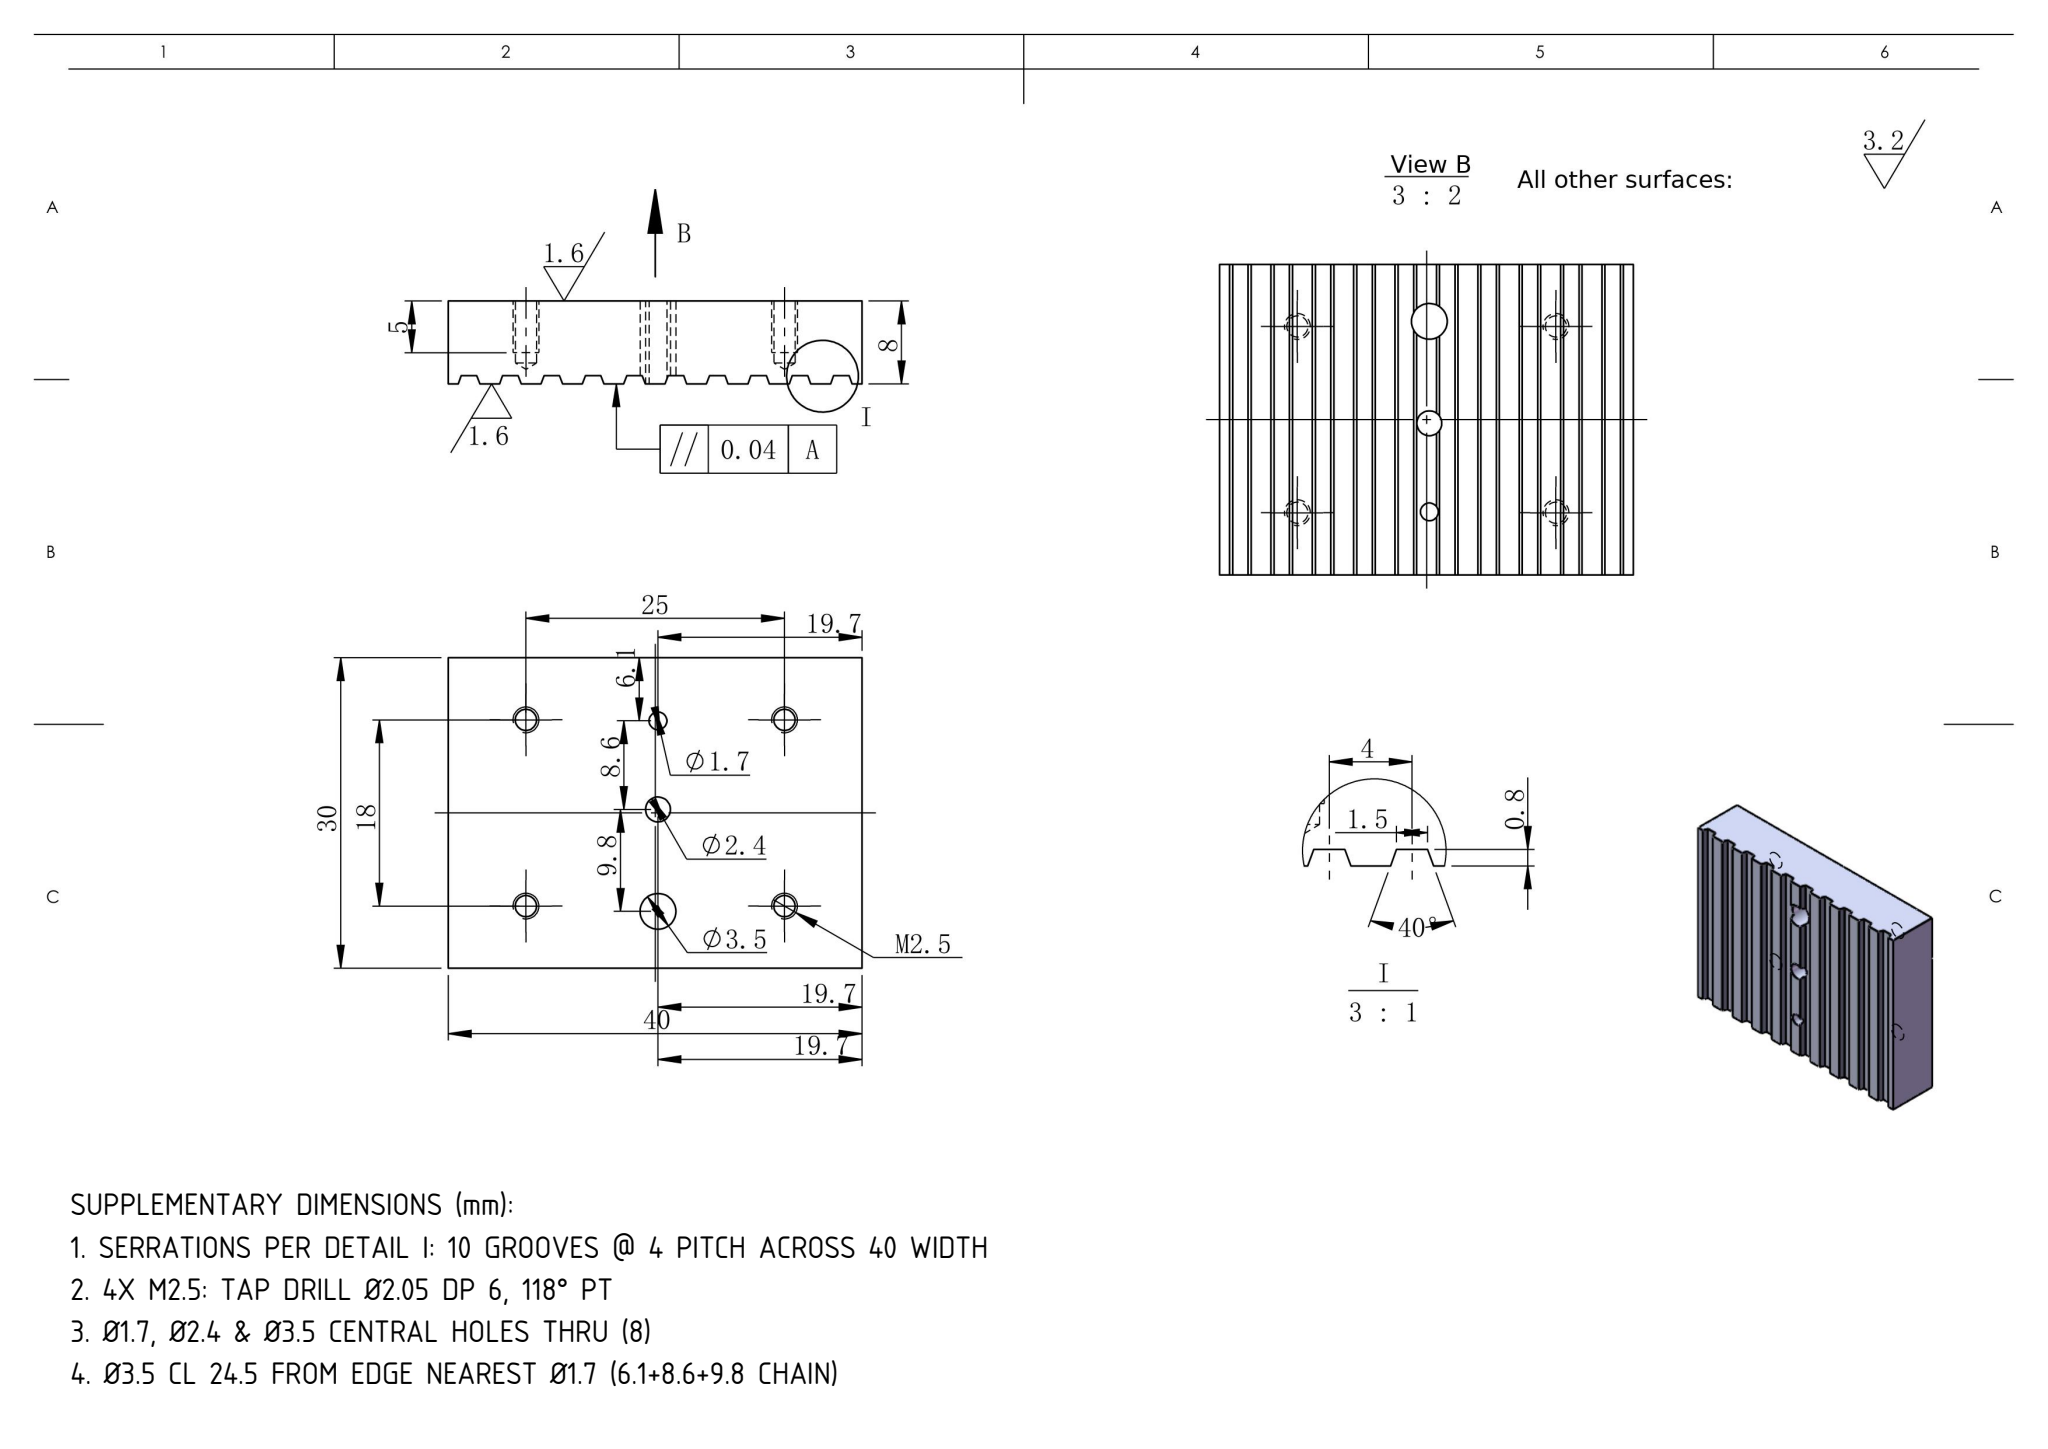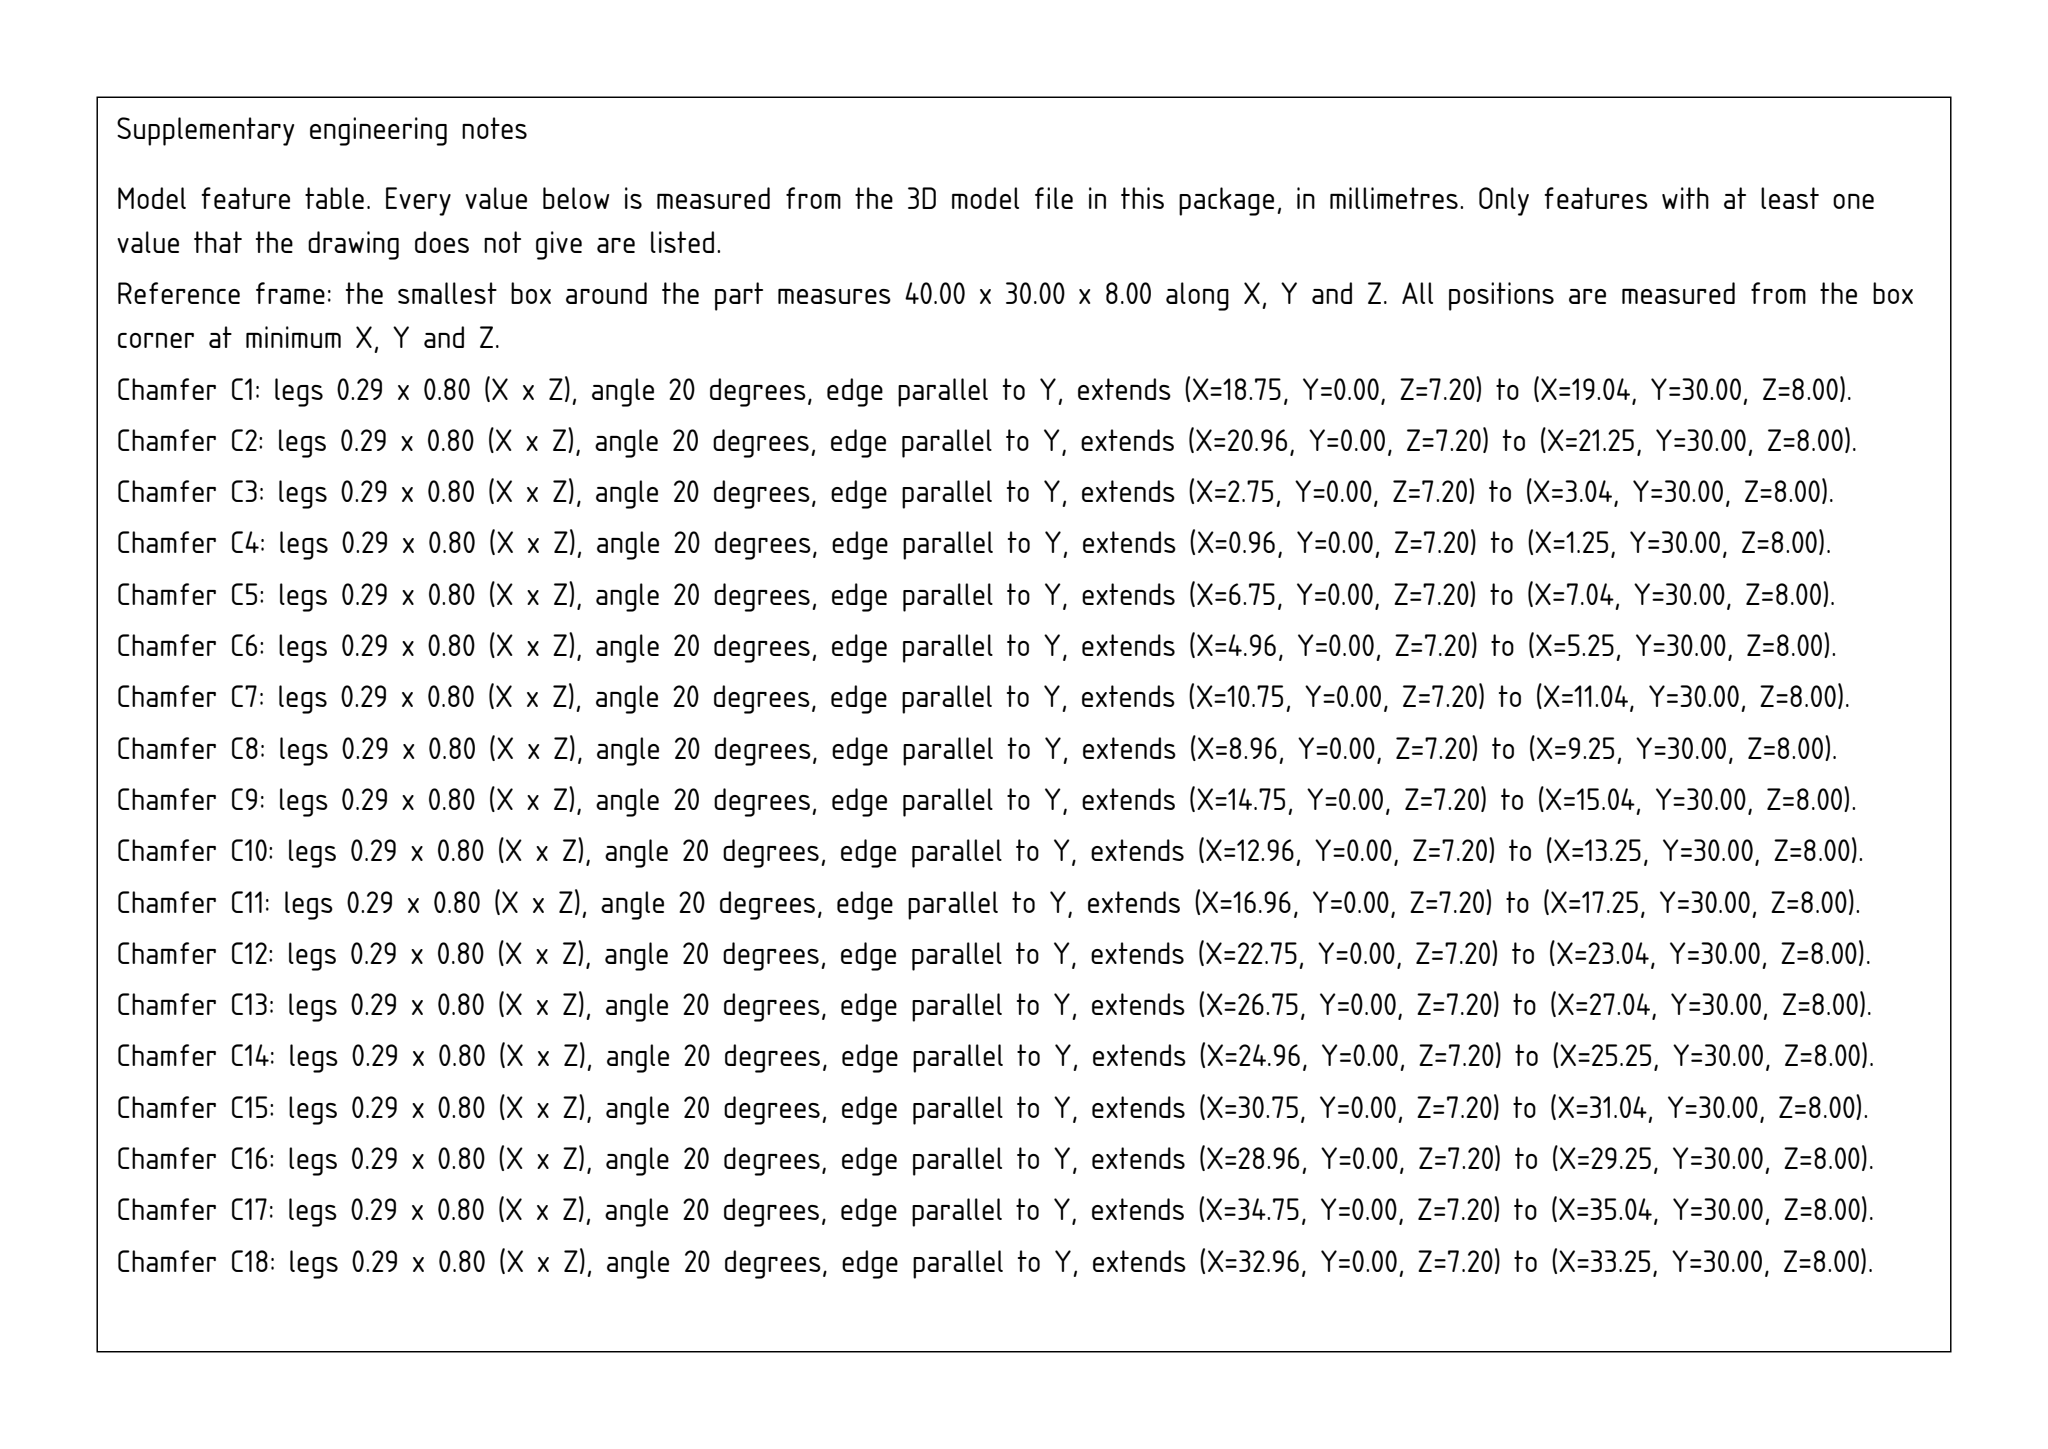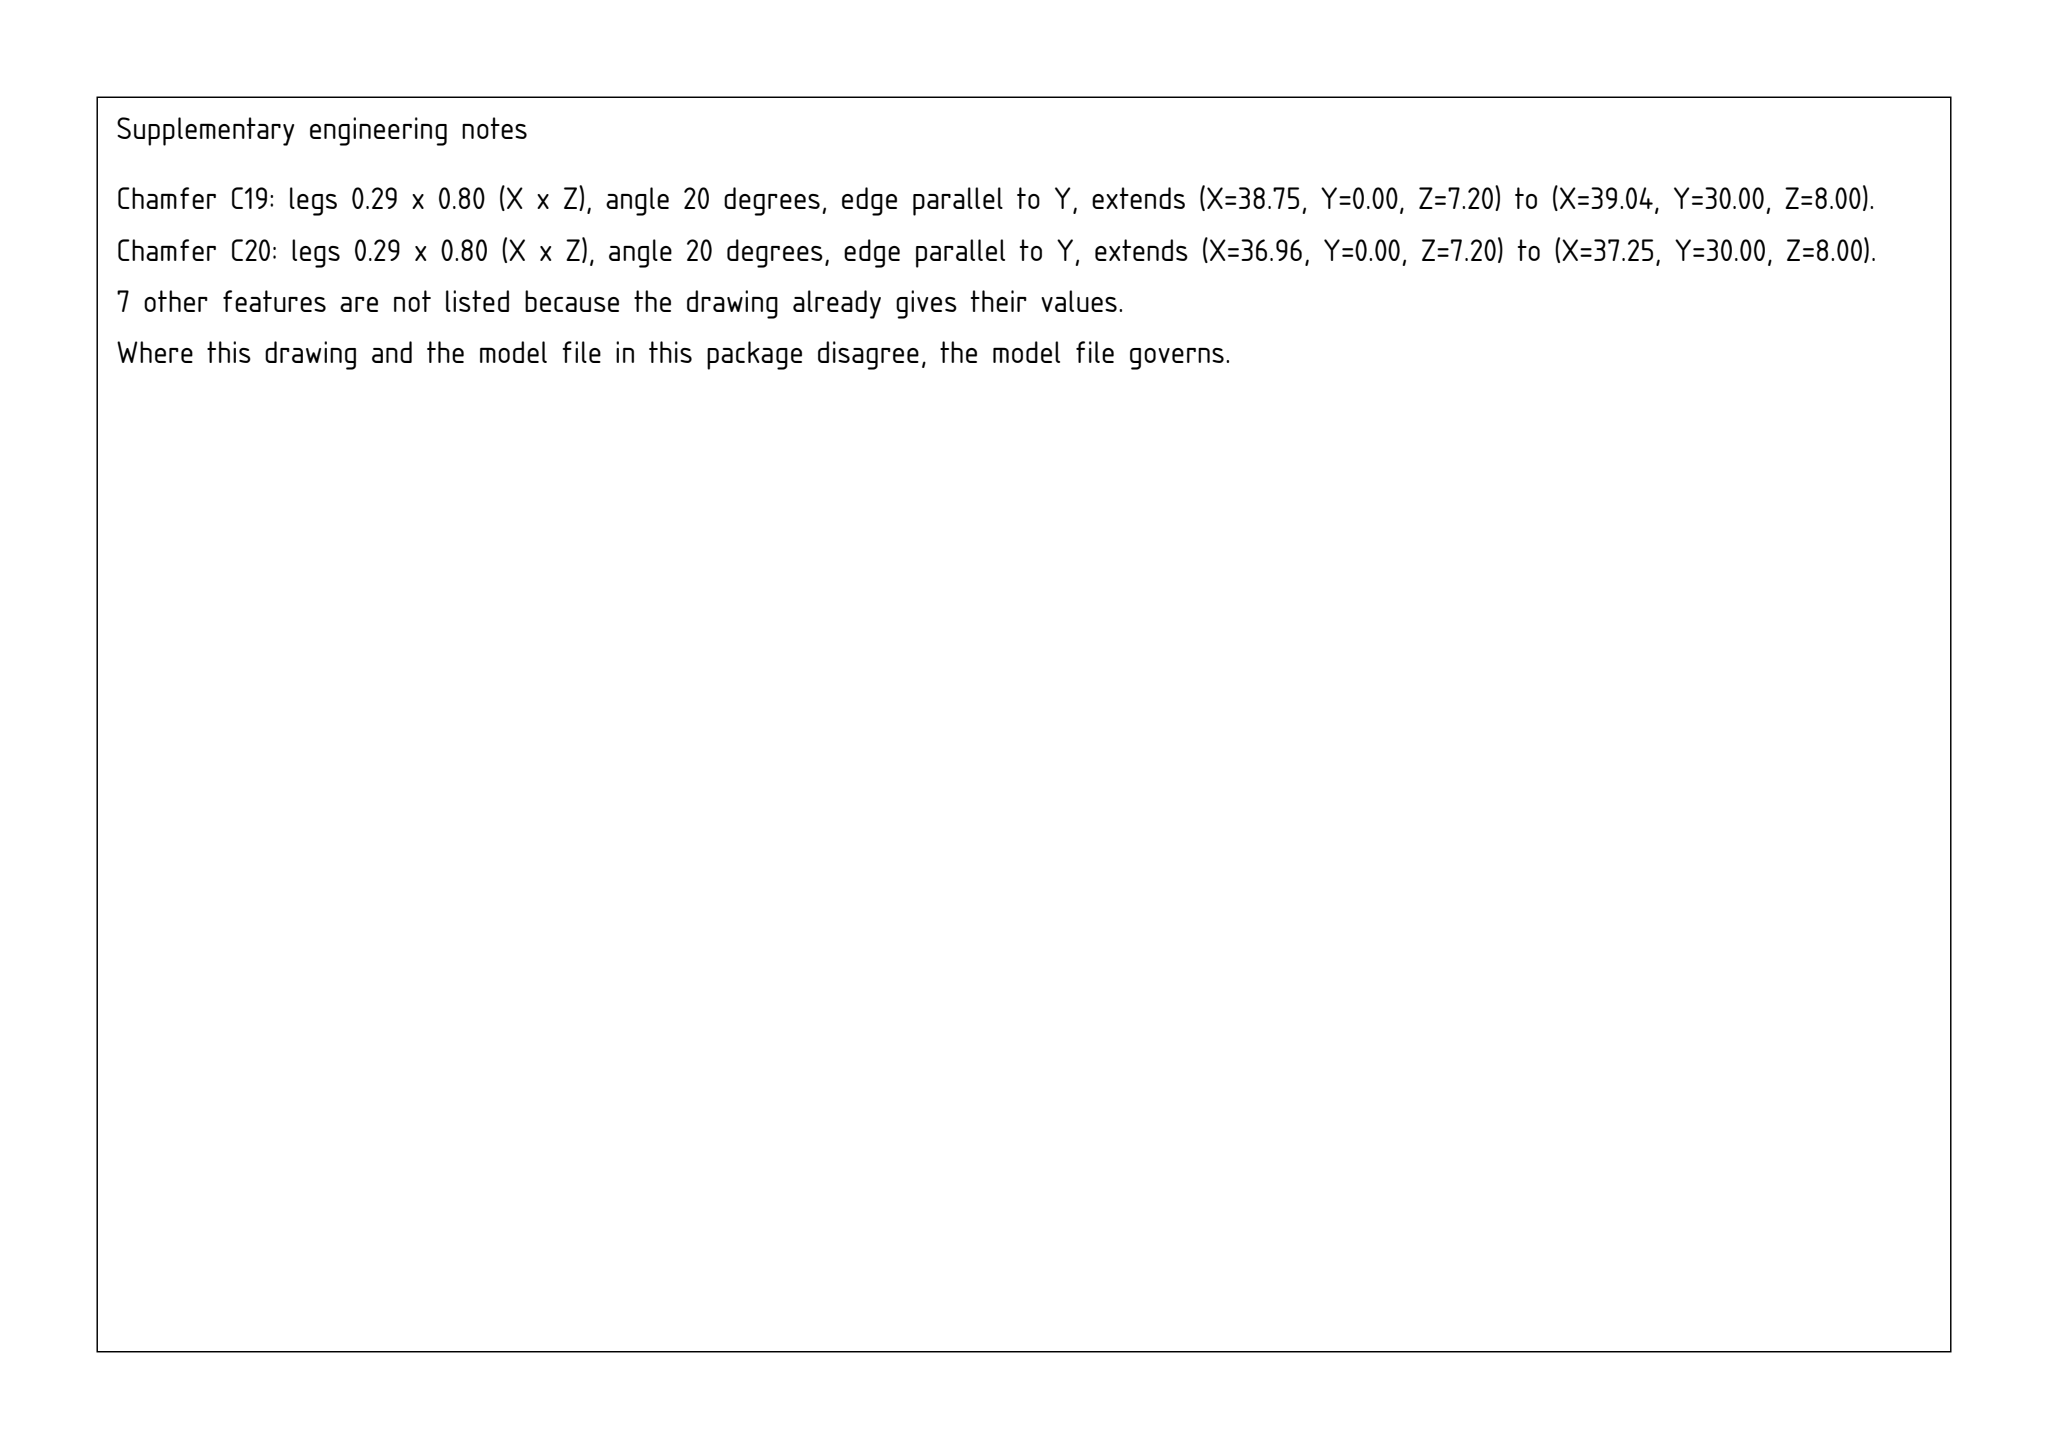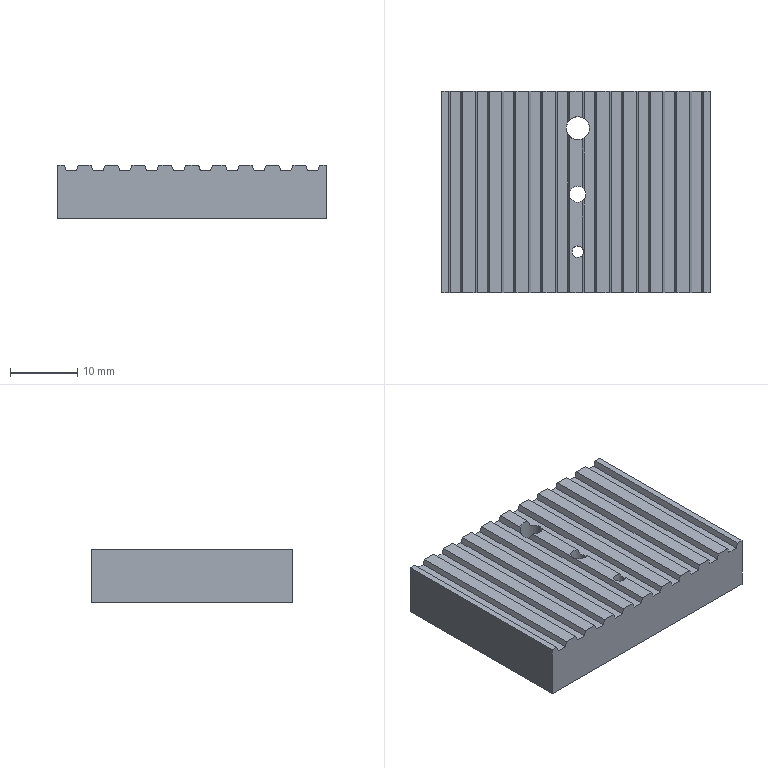Part | SolidWorks | mm | 1 solid | 72 faces | box 40 x 30 x 8 mm | volume 8960 mm3 | plane 50 | cylinder 14 | cone 8 | commonest cylinder face diameters 2.05 x8 3.459 x2 1.724 x2 2.409 x2
build123d program:
from build123d import *

# Parameters (mm, degrees)
SKETCH1_W               = 40
SKETCH1_H               = 30
EXTRUDE1_DEPTH          = 8
CUT_EXTRUDE1_DEPTH      = 51.636
LPATTERN1_COUNT         = 10
LPATTERN1_PITCH         = 4
M2_5_TAPPED_HOLE1_D     = 2.05
M2_5_TAPPED_HOLE1_DEPTH = 6
M2_5_TAPPED_HOLE1_TIP   = 0.6159
SKETCH6_R               = 1.73
SKETCH6_R_2             = 0.862
SKETCH6_R_3             = 1.204
CUT_EXTRUDE2_DEPTH      = 10


with BuildPart() as part:
    # Sketch1 → Extrude1 (new body)
    with BuildSketch(Plane.XY):
        with Locations((20, 15)):
            Rectangle(SKETCH1_W, SKETCH1_H)
    extrude(amount=EXTRUDE1_DEPTH)

    # Sketch3 → Cut-Extrude1 (cut, through all)
    with BuildSketch(Plane.XZ):
        Polygon((0.9588, 8), (1.25, 7.2), (2.75, 7.2), (3.041, 8), align=None)
    cut_extrude1 = extrude(amount=-CUT_EXTRUDE1_DEPTH, mode=Mode.SUBTRACT)

    # LPattern1: Cut-Extrude1 ×10
    with Locations(*[(i * LPATTERN1_PITCH, 0, 0) for i in range(1, LPATTERN1_COUNT)]):
        add(cut_extrude1, mode=Mode.SUBTRACT)

    # M2.5 Tapped Hole1
    with Locations(Plane(origin=(0, 0, 0), x_dir=(-1, 0, 0), z_dir=(0, 0, -1))):
        with Locations((-32.5, 24), (-7.5, 24), (-7.5, 6), (-32.5, 6)):
            Hole(M2_5_TAPPED_HOLE1_D / 2, depth=M2_5_TAPPED_HOLE1_DEPTH)
            with Locations((0, 0, -(M2_5_TAPPED_HOLE1_DEPTH + M2_5_TAPPED_HOLE1_TIP / 2))):  # 118° drill point
                Cone(0, M2_5_TAPPED_HOLE1_D / 2, M2_5_TAPPED_HOLE1_TIP, mode=Mode.SUBTRACT)

    # Sketch6 → Cut-Extrude2 (cut)
    with BuildSketch(Plane(origin=(0, 0, 0), x_dir=(-1, 0, 0), z_dir=(0, 0, -1))):
        with Locations((-20.269, 24.505)):
            Circle(SKETCH6_R)
        with Locations((-20.269, 6.093)):
            Circle(SKETCH6_R_2)
        with Locations((-20.269, 14.656)):
            Circle(SKETCH6_R_3)
    extrude(amount=-CUT_EXTRUDE2_DEPTH, mode=Mode.SUBTRACT)


solid = part.part